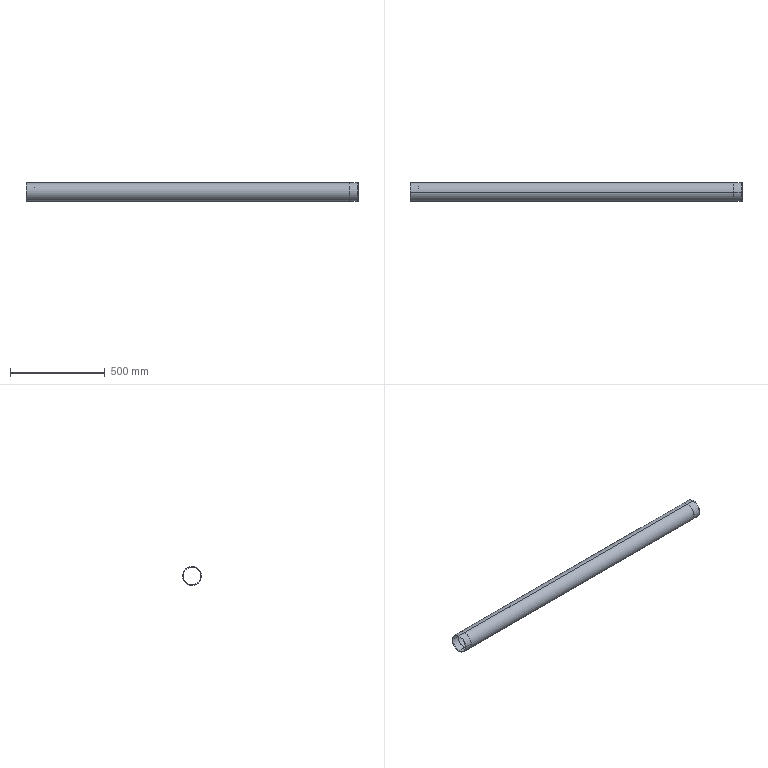Component | SolidWorks | 216InnerTubeAssembly-1_InnerTube-1 | 1 solid | 18 faces | box 1750 x 98.8 x 98.8 mm | volume 1502105 mm3 | cylinder 12 | plane 6 | commonest cylinder face diameters 96 x4 96.01 x2 98.8 x2 98 x2 93 x2 | material Alloy Steel
build123d program:
from build123d import *

# Parameters (mm, degrees)
SKETCH1_W = 41.278
SKETCH1_H = 2.005


with BuildPart() as part:
    # Model → Revolve1 (revolve)
    with BuildSketch(Plane.XY, mode=Mode.PRIVATE) as revolve1_sk:
        Polygon((0, 48), (0, 49.4), (1705, 49.4), (1705, 49), (1746, 49), (1746, 48), (1750, 48), (1750, 46.5), (45, 46.5), (45, 46.8), (4, 46.8), (4, 48), align=None)
    revolve(revolve1_sk.sketch.rotate(Axis((0.000009765, 0, 0), (1, 0, 0)), 90), axis=Axis((0.000009765, 0, 0), (1, 0, 0)))

    # Sketch1 → Cut-Revolve1 (revolve, cut)
    with BuildSketch(Plane.XY, mode=Mode.PRIVATE) as cut_revolve1_sk:
        with Locations((24.361, 47.002)):
            Rectangle(SKETCH1_W, SKETCH1_H)
    revolve(cut_revolve1_sk.sketch.rotate(Axis((-1.278, 0, 0), (1, 0, 0)), 90), axis=Axis((-1.278, 0, 0), (1, 0, 0)), mode=Mode.SUBTRACT)


solid = part.part

# Placed as in the assembly
solid = solid.moved(Location((1143.278, 0, 0), (0, 0, 0)))